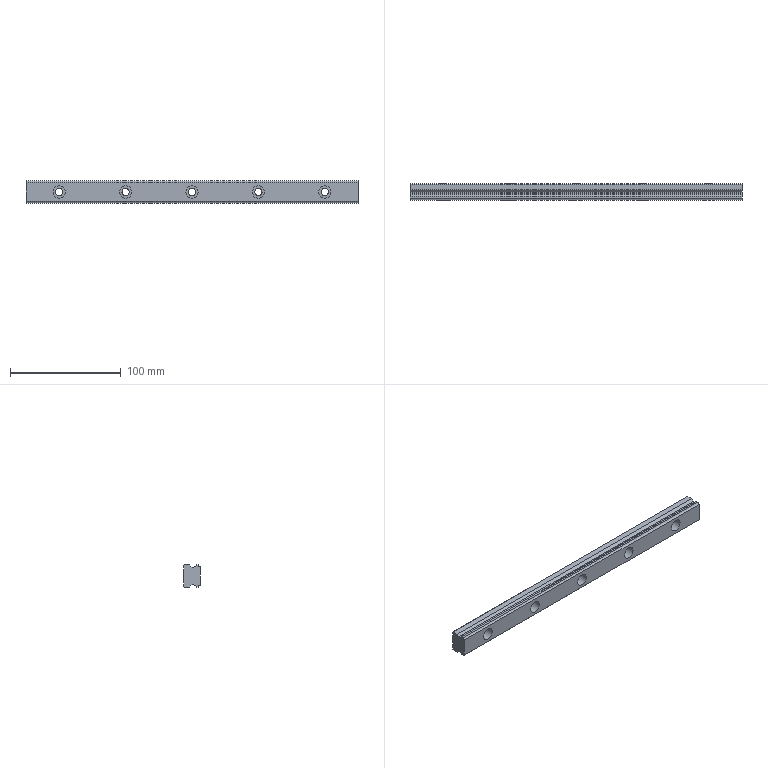Component | NX | GUIDE_RAIL_1 | 1 solid | 39 faces | volume 77461 mm3 | plane 25 | cylinder 14 | commonest cylinder face diameters 6.6 x5 11 x5 3.5 x4